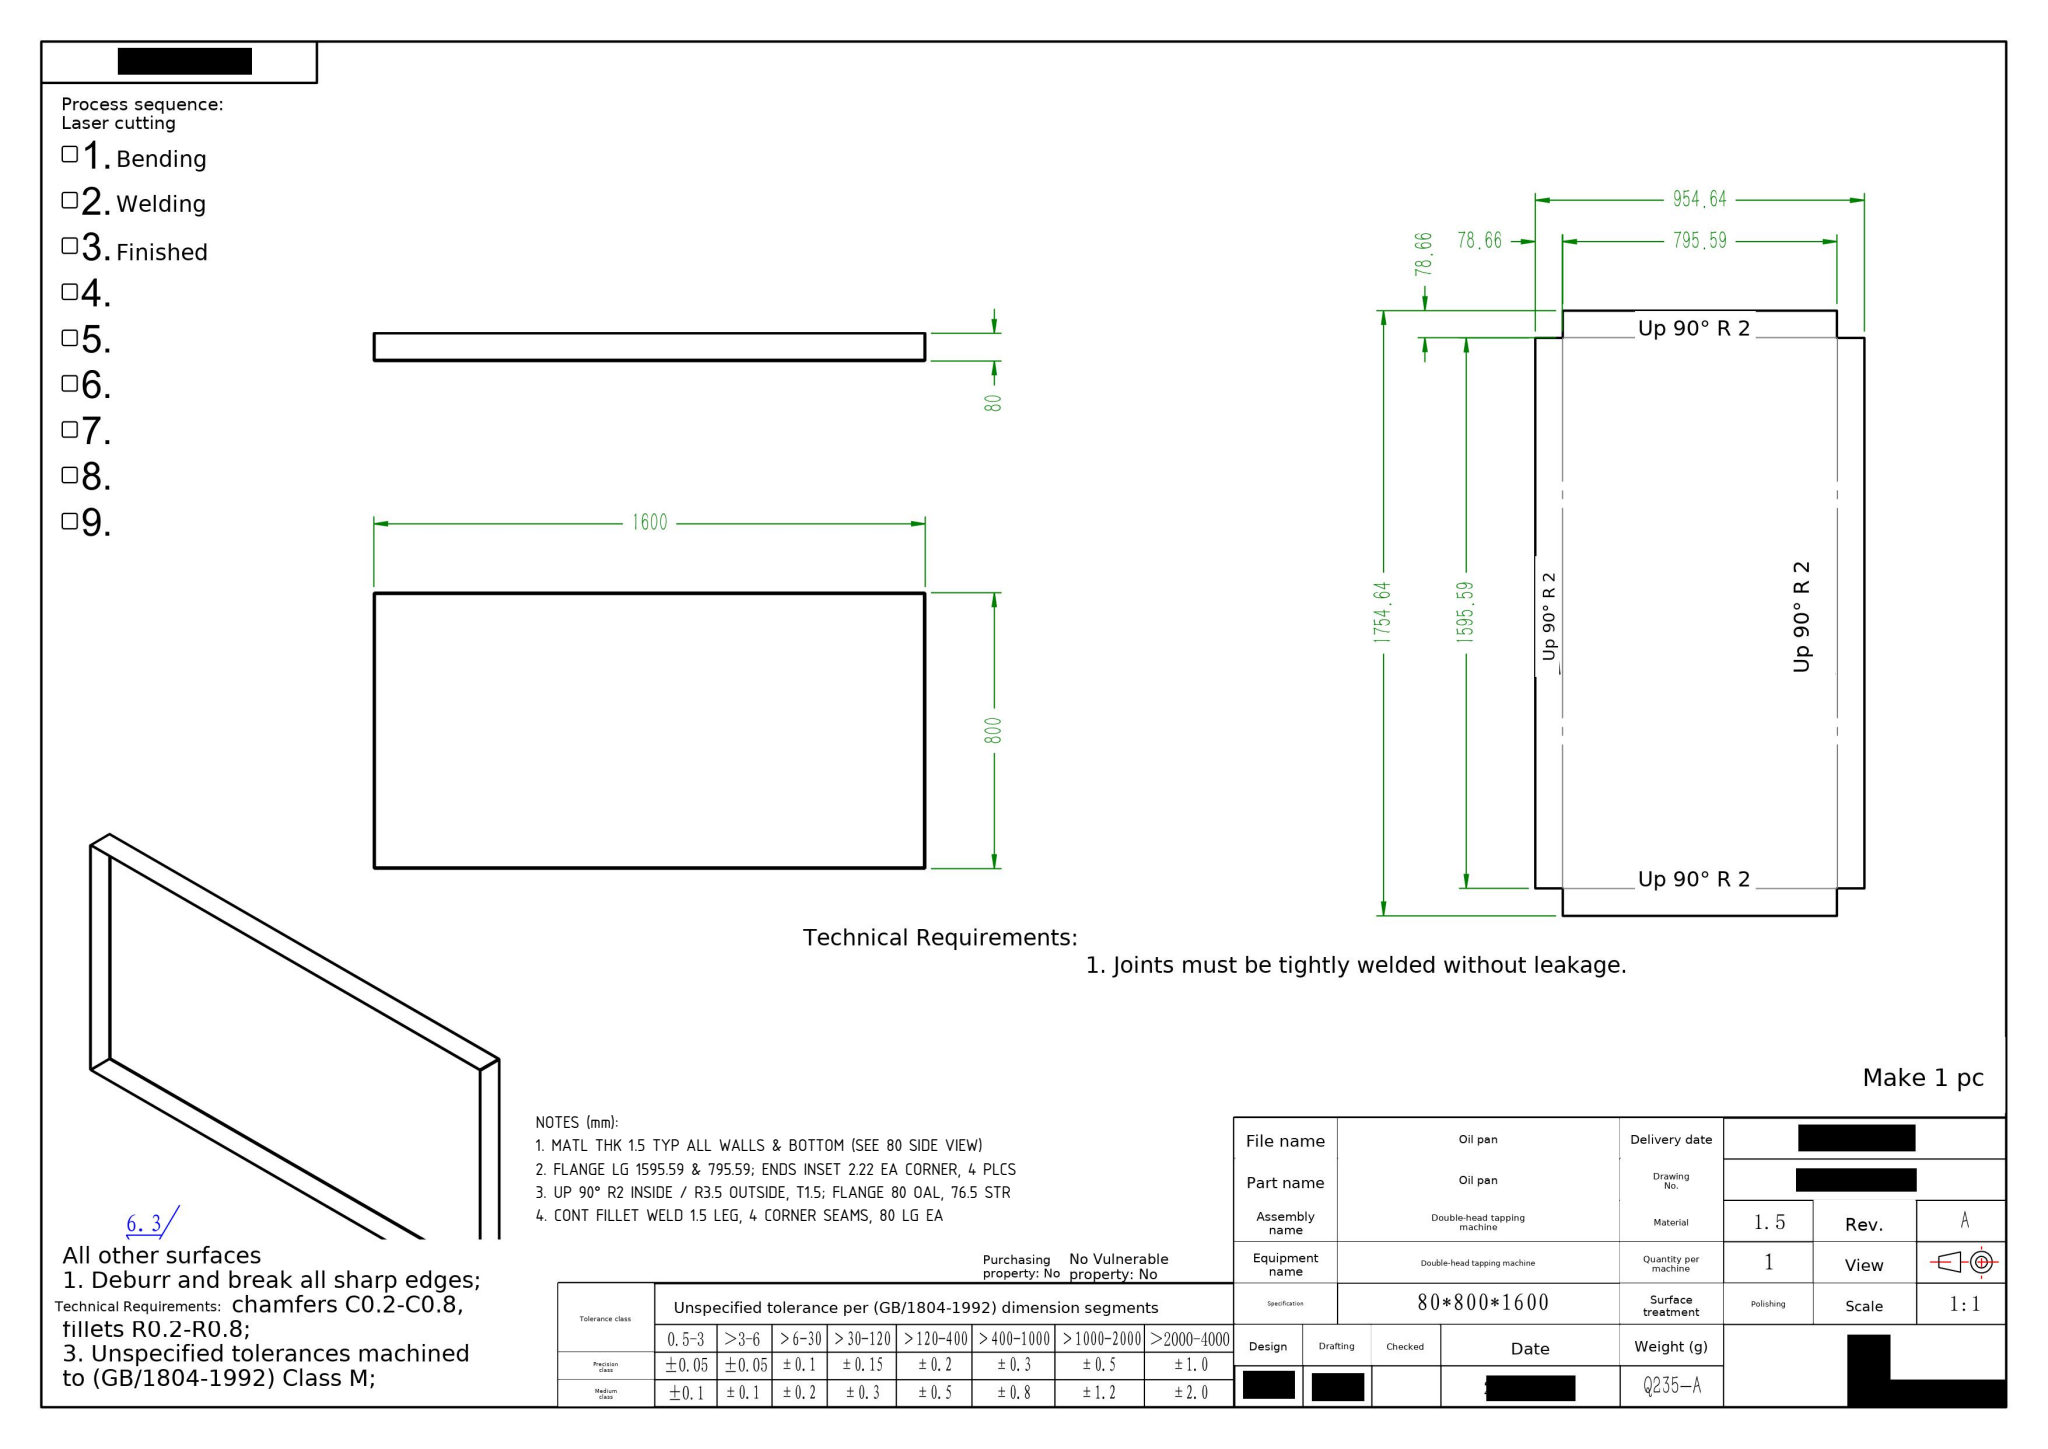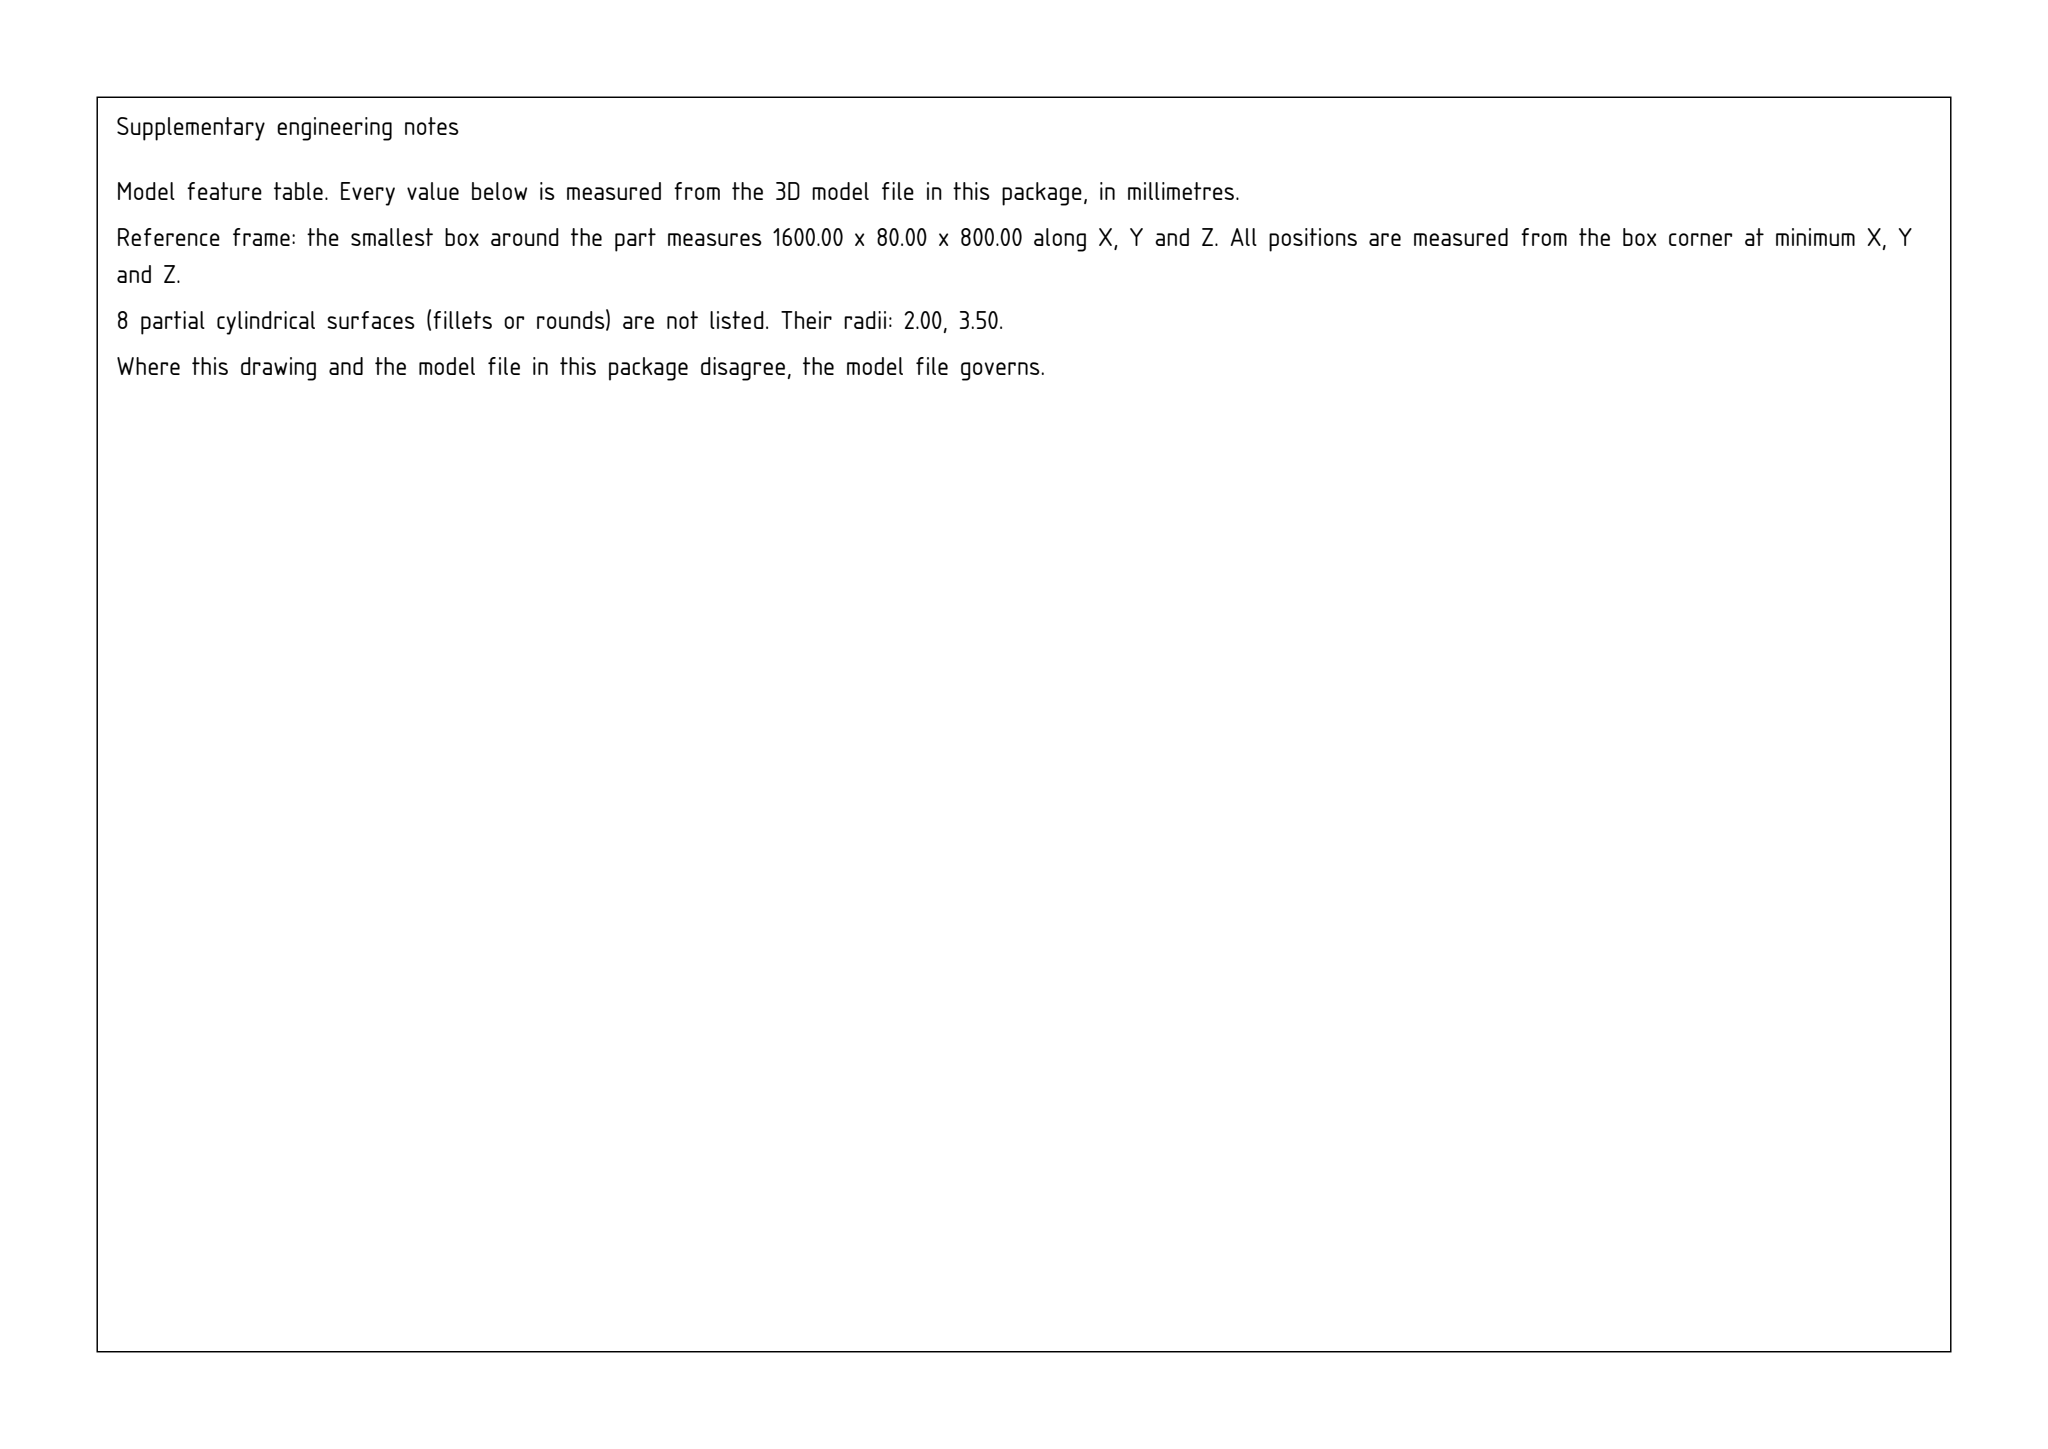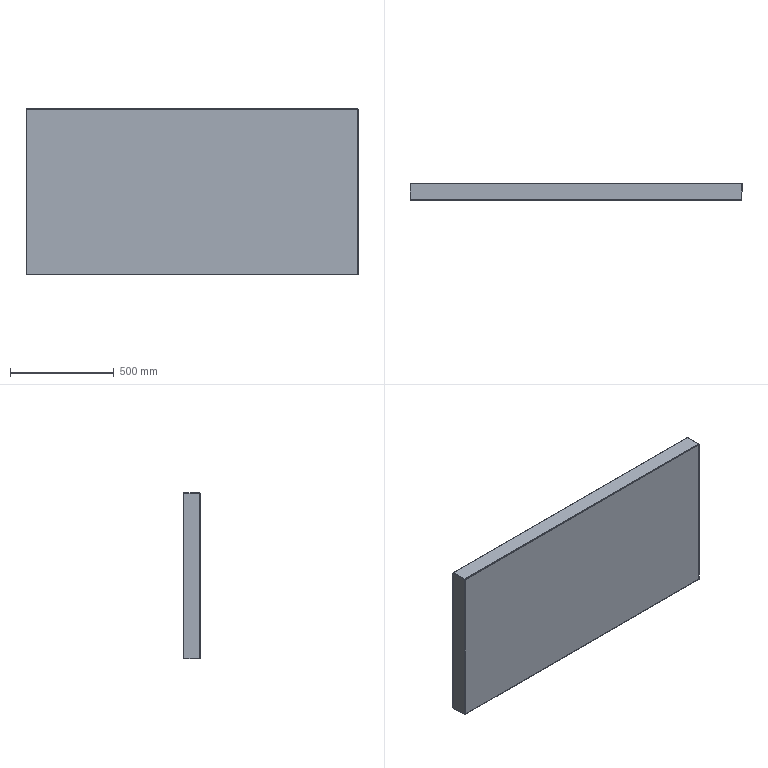Part | SolidWorks | mm | 1 solid | 38 faces | box 1600 x 80 x 800 mm | volume 2474601 mm3 | plane 22 | spline 8 | cylinder 8 | commonest cylinder face diameters 7 x4 4 x4
Drawing notes:
MATL THK 1.5 TYP ALL WALLS & BOTTOM (SEE 80 SIDE VIEW) | from the solid: Parallel face pairs y=0.02/1.52, x=0.02/1.52, x=1598.52/1600.02 => t=1.5
FLANGE LG 1595.59 & 795.59; ENDS INSET 2.22 EA CORNER, 4 PLCS | from the solid: Bend cyl lengths 1595.59 (x-axis) & 795.59 (z-axis); end planes x=2.22/1597.81, z=2.22/797.81 vs bbox 1600.03 x 800.03
UP 90° R2 INSIDE / R3.5 OUTSIDE, T1.5; FLANGE 80 OAL, 76.5 STR | from the solid: Bend cyls Ø4 (R2 inner) & Ø7 (R3.5 outer) at 3.52,3.52; bbox y=80.015; 80.02-3.52=76.5 straight
CONT FILLET WELD 1.5 LEG, 4 CORNER SEAMS, 80 LG EA | from the solid: 0.70 open corner gap (flange end x=2.22 vs flange face x=1.52), seam full flange ht 80.015, t=1.5